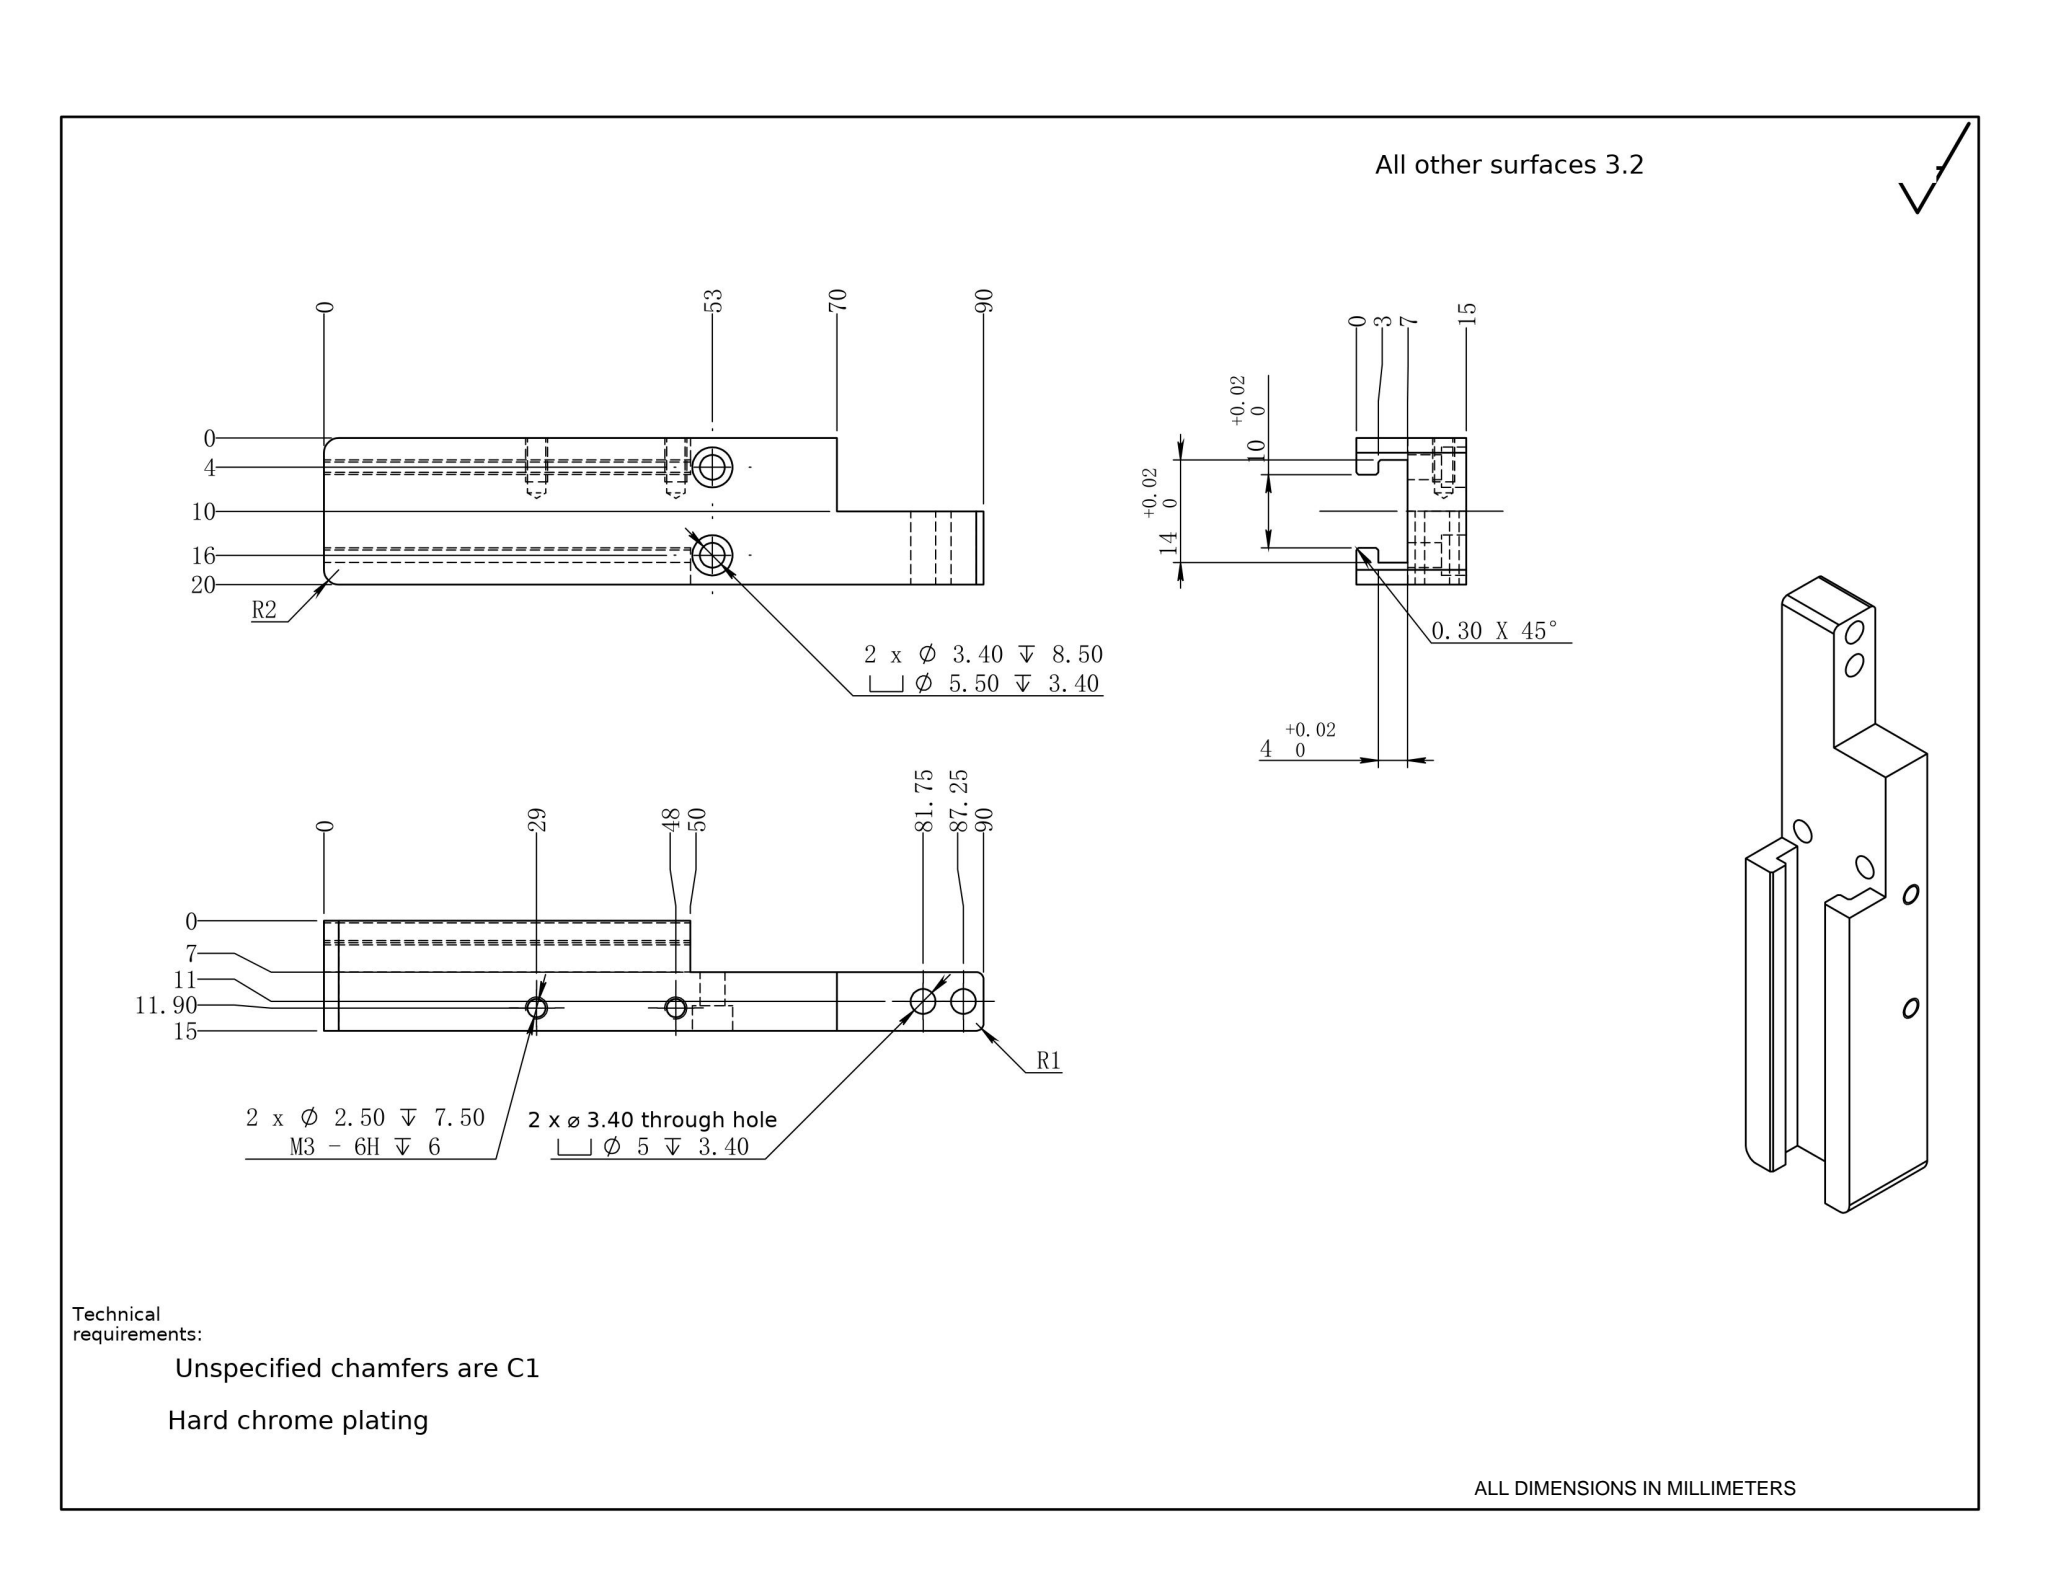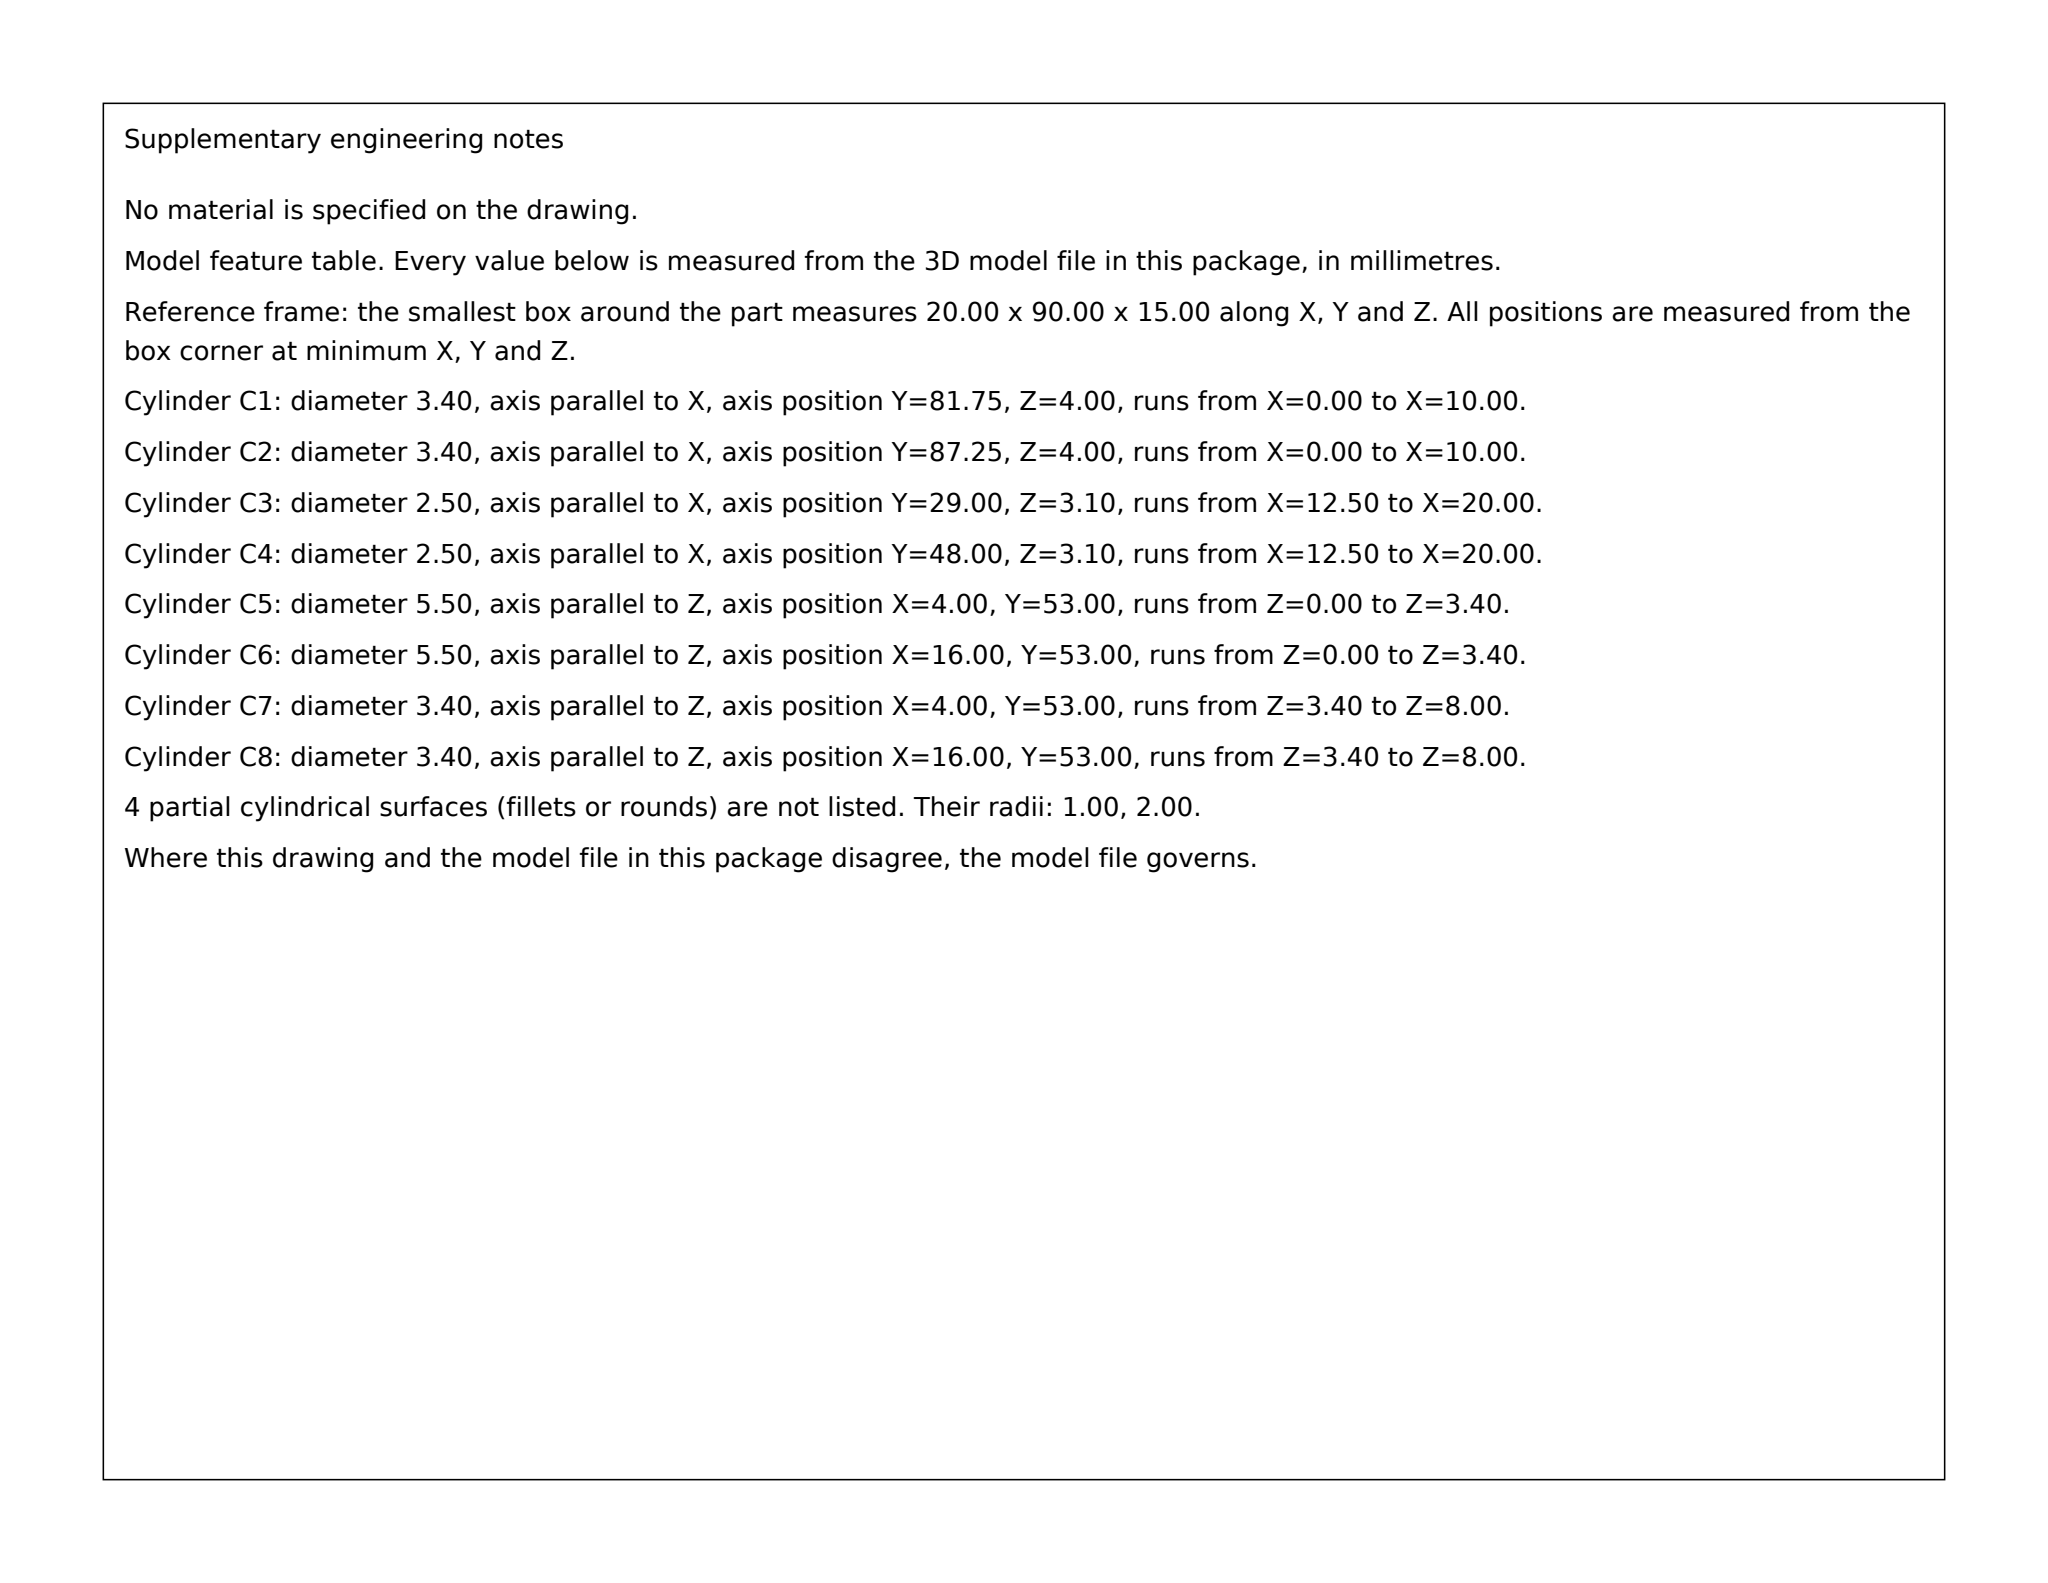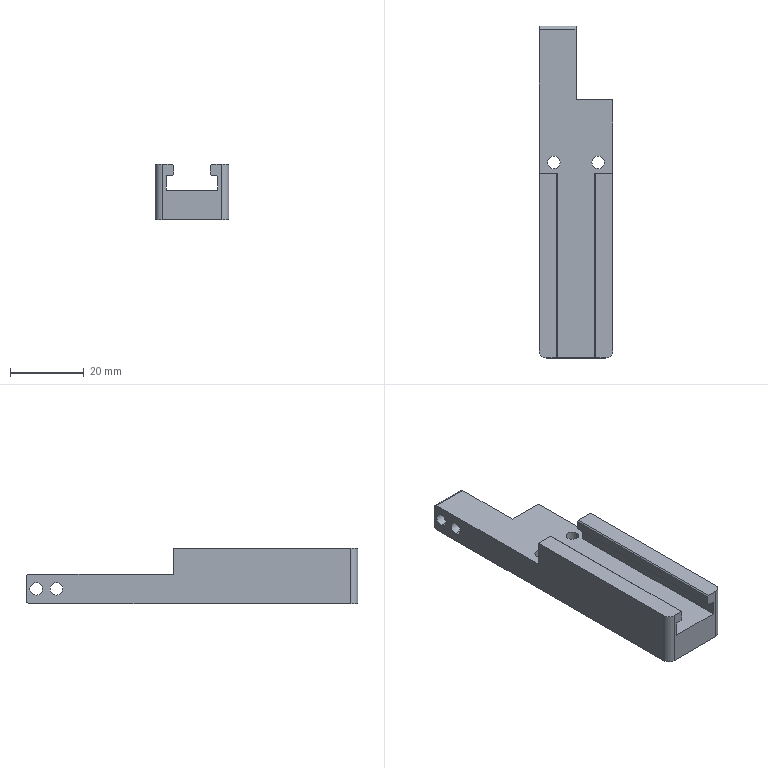Part | SolidWorks | mm | 1 solid | 49 faces | box 20 x 90 x 15 mm | volume 14960 mm3 | plane 25 | cylinder 20 | cone 4 | commonest cylinder face diameters 3.4 x8 2.5 x4 5.5 x4 2 x2 4 x2
build123d program:
from build123d import *

# Parameters (mm, degrees)
SKETCH1_W                                       = 20
SKETCH1_H                                       = 90
BOSS_EXTRUDE1_DEPTH                             = 15
SKETCH2_W                                       = 10
SKETCH2_H                                       = 6
CUT_EXTRUDE1_DEPTH                              = 92.788
SKETCH3_W                                       = 14
SKETCH3_H                                       = 4
CUT_EXTRUDE2_DEPTH                              = 92.788
SKETCH4_W                                       = 20
SKETCH4_H                                       = 40
CUT_EXTRUDE3_DEPTH                              = 47.787
M3_HEX_SOCKET_HEAD_CAP_SCREW_CBORE3_D           = 3.4
M3_HEX_SOCKET_HEAD_CAP_SCREW_CBORE3_DEPTH       = 8.5
M3_HEX_SOCKET_HEAD_CAP_SCREW_CBORE3_CBORE_D     = 5.5
M3_HEX_SOCKET_HEAD_CAP_SCREW_CBORE3_CBORE_DEPTH = 3.4
M3_HEX_SOCKET_HEAD_CAP_SCREW_CBORE3_TIP         = 1.021
M3_HEX_SOCKET_HEAD_CAP_SCREW_CBORE5_D           = 3.4
M3_HEX_SOCKET_HEAD_CAP_SCREW_CBORE5_CBORE_D     = 5
M3_HEX_SOCKET_HEAD_CAP_SCREW_CBORE5_CBORE_DEPTH = 3.4
FILLET1_R                                       = 1
CHAMFER1_SIZE                                   = 0.3
FILLET2_R                                       = 2
SKETCH11_W                                      = 10
SKETCH11_H                                      = 20
CUT_EXTRUDE4_DEPTH                              = 47.787
M3_TAPPED_HOLE1_D                               = 2.5
M3_TAPPED_HOLE1_DEPTH                           = 7.5
M3_TAPPED_HOLE1_TIP                             = 0.7511


with BuildPart() as part:
    # Sketch1 → Boss-Extrude1 (new body)
    with BuildSketch(Plane.XY):
        Rectangle(SKETCH1_W, SKETCH1_H)
    extrude(amount=BOSS_EXTRUDE1_DEPTH)

    # Sketch2 → Cut-Extrude1 (cut, through all)
    with BuildSketch(Plane(origin=(0, 45, 0), x_dir=(1, 0, 0), z_dir=(0, 1, 0))):
        with Locations((0, -15)):
            Rectangle(SKETCH2_W, SKETCH2_H)
    extrude(amount=-CUT_EXTRUDE1_DEPTH, mode=Mode.SUBTRACT)

    # Sketch3 → Cut-Extrude2 (cut, through all)
    with BuildSketch(Plane(origin=(0, 45, 0), x_dir=(1, 0, 0), z_dir=(0, 1, 0))):
        with Locations((0, -10)):
            Rectangle(SKETCH3_W, SKETCH3_H)
    extrude(amount=-CUT_EXTRUDE2_DEPTH, mode=Mode.SUBTRACT)

    # Sketch4 → Cut-Extrude3 (cut, through all)
    with BuildSketch(Plane.XY.offset(8)):
        with Locations((0, 25)):
            Rectangle(SKETCH4_W, SKETCH4_H)
    extrude(amount=CUT_EXTRUDE3_DEPTH, mode=Mode.SUBTRACT)

    # M3 Hex Socket Head Cap Screw CBORE3
    with Locations(Plane(origin=(0, 0, 0), x_dir=(-1, 0, 0), z_dir=(0, 0, -1))):
        with Locations((-6, 8), (6, 8)):
            CounterBoreHole(M3_HEX_SOCKET_HEAD_CAP_SCREW_CBORE3_D / 2, M3_HEX_SOCKET_HEAD_CAP_SCREW_CBORE3_CBORE_D / 2, M3_HEX_SOCKET_HEAD_CAP_SCREW_CBORE3_CBORE_DEPTH, depth=M3_HEX_SOCKET_HEAD_CAP_SCREW_CBORE3_DEPTH)
            with Locations((0, 0, -(M3_HEX_SOCKET_HEAD_CAP_SCREW_CBORE3_DEPTH + M3_HEX_SOCKET_HEAD_CAP_SCREW_CBORE3_TIP / 2))):  # 118° drill point
                Cone(0, M3_HEX_SOCKET_HEAD_CAP_SCREW_CBORE3_D / 2, M3_HEX_SOCKET_HEAD_CAP_SCREW_CBORE3_TIP, mode=Mode.SUBTRACT)

    # M3 Hex Socket Head Cap Screw CBORE5 (through all)
    with Locations(Plane(origin=(10, 0, 0), x_dir=(0, 0, -1), z_dir=(1, 0, 0))):
        with Locations((-4, 42.25), (-4, 36.75)):
            CounterBoreHole(M3_HEX_SOCKET_HEAD_CAP_SCREW_CBORE5_D / 2, M3_HEX_SOCKET_HEAD_CAP_SCREW_CBORE5_CBORE_D / 2, M3_HEX_SOCKET_HEAD_CAP_SCREW_CBORE5_CBORE_DEPTH)

    # Fillet1
    fillet1_edges = [part.edges().sort_by_distance(p)[0] for p in [
        (0, 45, 8),
        (0, 45, 0),
    ]]
    fillet(fillet1_edges, radius=FILLET1_R)

    # Chamfer1
    chamfer1_edges = [part.edges().sort_by_distance(p)[0] for p in [
        (-5, -20, 15),
        (5, -20, 12),
        (-5, -20, 12),
        (7, -20, 12),
        (5, -20, 15),
    ]]
    chamfer(chamfer1_edges, length=CHAMFER1_SIZE)

    # Fillet2
    fillet2_edges = [part.edges().sort_by_distance(p)[0] for p in [
        (10, -45, 7.5),
        (-10, -45, 7.5),
    ]]
    fillet(fillet2_edges, radius=FILLET2_R)

    # Sketch11 → Cut-Extrude4 (cut, through all)
    with BuildSketch(Plane.XY.offset(8)):
        with Locations((5, 35)):
            Rectangle(SKETCH11_W, SKETCH11_H)
    extrude(amount=-CUT_EXTRUDE4_DEPTH, mode=Mode.SUBTRACT)

    # M3 Tapped Hole1
    with Locations(Plane(origin=(10, 0, 0), x_dir=(0, 0, -1), z_dir=(1, 0, 0))):
        with Locations((-3.1, 3), (-3.1, -16)):
            Hole(M3_TAPPED_HOLE1_D / 2, depth=M3_TAPPED_HOLE1_DEPTH)
            with Locations((0, 0, -(M3_TAPPED_HOLE1_DEPTH + M3_TAPPED_HOLE1_TIP / 2))):  # 118° drill point
                Cone(0, M3_TAPPED_HOLE1_D / 2, M3_TAPPED_HOLE1_TIP, mode=Mode.SUBTRACT)


solid = part.part